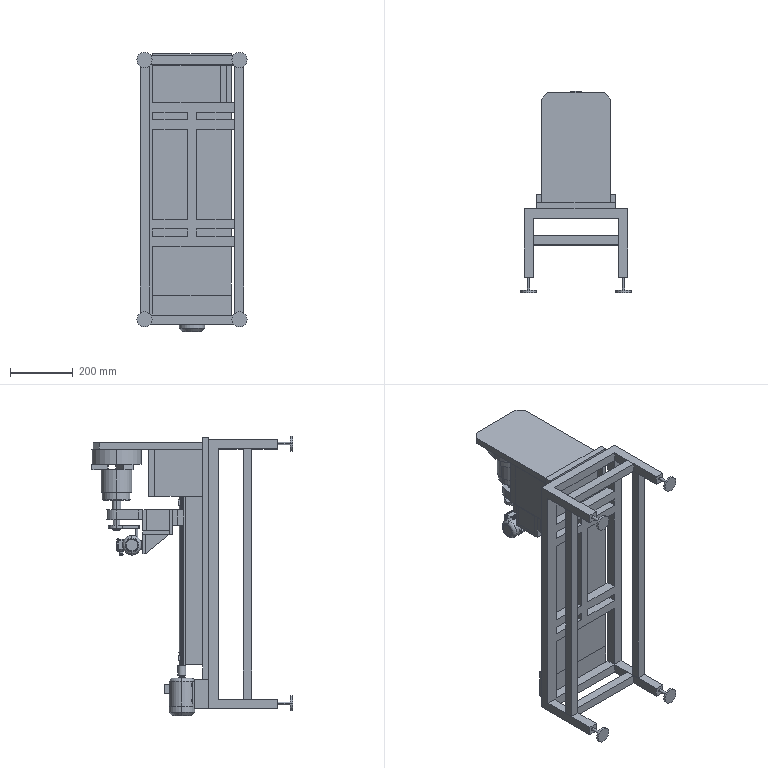Assembly | SolidWorks | mm | 29 component files | 64 solids | 2723 faces | box 351.7 x 642.03 x 891.18 mm | volume 19068992 mm3 | plane 1496 | cylinder 842 | spline 199 | cone 180 | torus 6 | commonest cylinder face diameters 5 x129 1 x116 2 x95 0.5 x65 3 x54 2.5 x27 6 x20 10 x18
Bill of materials:
BearingHousing | 1 |  | T-shaped bracket: a flat lug with a rounded end and one large through-hole, joined at right angles to a rectangular base bar that has two small through-holes.
BearingHousingFloor | 1 |  | Open-topped rectangular box-like housing. It has a thin-walled cavity, two stacked lugs with round holes sticking out from one side, a sloped flange extension with small holes on the opposite side, and stepped notches in the outline.
Belt | 1 |  | Thin-walled closed band or loop shaped like a teardrop. It has a large rounded end, a small rounded end and two straight tapering sides, with a short uniform height.
Chuck | 1 |  | Round disc with a small central through-bore. On one face is a stepped boss with split, chamfered prongs, and the bore wall shows a ridged or serrated pattern.
ChuckHolder | 1 |  | Thin sheet-like bracket: a tall flat plate with a horizontal flange at the top, a rectangular block under the flange, small side tabs, and chamfered top corners.
Coupling | 1 |  | Thick-walled cylindrical sleeve or bushing with a round through-bore and one rectangular keyway along the length of the bore.
DriveAxis | 1 |  | Slender stepped cylindrical pin or shaft: two sections of slightly different diameter, with a small rectangular slot or keyway at one end.
DriveMotor | 1 |  | Simplified cylindrical body with a domed end cap, a protruding stepped shaft, two mounting feet and a rectangular block on top. The overall envelope looks like an electric motor.
FixedFrame | 1 |  | Plain solid rectangular block (cuboid) with sharp edges and no visible holes or features.
Frame | 1 |  | Tall rectangular open frame made of square-section members, with intermediate crossbars and a central upright. It stands on four leveling-type feet, each a disc pad on a short stem.
GearedMotor | 1 |  | Detailed, roughly modelled assembly-like body: a ribbed cylindrical housing with a domed end cover and a rectangular box on top, joined through a flange to a compact angular housing that has a keyed hollow bore. The overall look resembles a motor coupled to a right-angle gearbox.
GuideRail | 1 |  | Long straight bar with a symmetric profile: V-shaped notches on both sides and rounded corners, with a row of evenly spaced small holes along one face.
LeadScrew | 1 |  | Long, slender cylindrical shaft. Both ends step down to a short section of smaller diameter.
MirrorGuideRail | 1 |  | Long straight bar with a constant cross-section. A single evenly spaced row of small holes runs along its length. The cross-section has the same notch on both sides and rounded top corners.
MirrorSlider | 1 |  | Rectangular block with a channel running all the way through it, open on the underside. The channel's internal profile has notches on both sides with rounded corners.
PolishingAxis | 1 |  | Short cylindrical pin with a raised collar of larger diameter near one end and chamfers on both ends.
PolishingHead | 1 |  | Thick circular disc with a small central through hole and a chamfer on one outer edge.
Pulley | 1 |  | Rectangular block with a channel running all the way through it, open on the underside. The channel's internal profile has notches on both sides with rounded corners.
Slider | 1 |  | Flat circular ring, like a plain washer, with a large central hole and square-edged faces.
SmallWheel | 1 |  | Thick-walled cylindrical collar or hub with a central round bore and a single rectangular keyway slot.
TRCBASHexagonThroughHoleBolt[TRCBAS3-10] | 4 |  | Hexagonal-head bolt-like part with a long plain cylindrical shank and a chamfered tip.
TRCBASHexagonThroughHoleBolt[TRCBAS5-10] | 4 |  | Hexagonal-head bolt-like part with a shorter plain cylindrical shank and a chamfered tip.
Workpiece | 1 |  | Thin-walled cylindrical tube or sleeve, open at both ends.
Mates:
1. coincident | Pulley-1 face at (0, 0, -195) dir (0, 0, 1) | SmallWheel-1 face at (48.507, -64.609, -195) dir (0, 0, 1)
2. concentric | LeadScrew-1 face at (0, -208.707, -601) dir (0, 0, -1) r 8 | DriveMotor-1 face at (0, -208.707, -654.301) dir (0, 0, -1) r 5.5
3. concentric | DriveMotor-1 face at (0, -208.707, -654.301) dir (0, 0, -1) r 5.5 | Coupling-1 face at (0, -208.707, -643.144) dir (0, 0, -1) r 12.5
4. coincident | DriveMotor-1 face at (1.5, -209.324, -655.301) dir (1, 0, 0) | Coupling-1 face at (1.5, -205.207, -653.144) dir (-1, 0, 0)
5. distance | DriveMotor-1 face at (19.858, -243.43, -695.801) dir (0, 0, 1) | FixedFrame-1 face at (125, -251.035, -685.801) dir (0, 0, 1)
6. concentric | SmallWheel-1 face at (48.507, -64.609, -205) dir (0, 0, 1) r 7.5 | GearedMotor-1 face at (48.507, -64.609, -274.5) dir (0, 0, 1) r 3.5
7. coincident | BearingHousingFloor-1 face at (68.507, -84.609, -286.341) dir (0, 1, 0) | GearedMotor-1 face at (58.507, -84.609, -272.25) dir (0, -1, 0)
8. concentric | GearedMotor-1 face at (48.507, -64.609, -274.5) dir (0, 0, 1) r 3.5 | DriveAxis-1 face at (48.507, -64.609, -242) dir (0, 0, -1) r 3.5
9. coincident | GearedMotor-1 face at (47.257, -61.339, -275) dir (1, 0, 0) | DriveAxis-1 face at (47.257, -62.109, -243.502) dir (1, 0, 0)
10. coincident | GearedMotor-1 face at (42.688, -58.79, -275) dir (0, 0, -1) | DriveAxis-1 face at (48.507, -64.609, -275) dir (0, 0, -1)
11. coincident | SmallWheel-1 face at (48.507, -64.609, -195) dir (0, 0, 1) | DriveAxis-1 face at (48.507, -64.609, -195) dir (0, 0, 1)
12. concentric | GearedMotor-1 face at (62.257, -81.609, -269.75) dir (0, -1, 0) r 1.625 | TRCBASHexagonThroughHoleBolt[TRCBAS3-10]-1 face at (62.257, -79.609, -269.75) dir (0, 1, 0) r 1.5
13. coincident | GearedMotor-1 face at (50.603, -81.609, -272.25) dir (0, 1, 0) | TRCBASHexagonThroughHoleBolt[TRCBAS3-10]-1 face at (65.003, -81.609, -269.608) dir (0, -1, 0)
14. concentric | GearedMotor-1 face at (34.757, -81.609, -269.75) dir (0, -1, 0) r 1.625 | TRCBASHexagonThroughHoleBolt[TRCBAS3-10]-2 face at (34.757, -79.609, -269.75) dir (0, 1, 0) r 1.5
15. coincident | GearedMotor-1 face at (31.257, -81.609, -272.25) dir (0, 1, 0) | TRCBASHexagonThroughHoleBolt[TRCBAS3-10]-2 face at (37.507, -81.609, -269.75) dir (0, -1, 0)
16. concentric | GearedMotor-1 face at (62.257, -81.609, -247.25) dir (0, -1, 0) r 1.625 | TRCBASHexagonThroughHoleBolt[TRCBAS3-10]-3 face at (62.257, -79.609, -247.25) dir (0, 1, 0) r 1.5
17. coincident | GearedMotor-1 face at (50.603, -81.609, -250.5) dir (0, 1, 0) | TRCBASHexagonThroughHoleBolt[TRCBAS3-10]-3 face at (65.003, -81.609, -247.108) dir (0, -1, 0)
18. concentric | GearedMotor-1 face at (34.757, -81.609, -247.25) dir (0, -1, 0) r 1.625 | TRCBASHexagonThroughHoleBolt[TRCBAS3-10]-4 face at (34.757, -79.609, -247.25) dir (0, 1, 0) r 1.5
19. coincident | GearedMotor-1 face at (31.257, -81.609, -250.5) dir (0, 1, 0) | TRCBASHexagonThroughHoleBolt[TRCBAS3-10]-4 face at (37.503, -81.609, -247.108) dir (0, -1, 0)
20. concentric | DriveMotor-1 edge at (31.25, -244.207, -754.301) dir (0, 1, 0) r 2.5 | TRCBASHexagonThroughHoleBolt[TRCBAS5-10]-1 face at (31.25, -240.707, -754.301) dir (0, 1, 0) r 2.5
21. parallel | DriveMotor-1 face at (27, -244.207, -763.301) dir (0, 1, 0) | FixedFrame-1 face at (0, -248.735, 48) dir (0, 1, 0)
22. coincident | DriveMotor-1 face at (27, -244.207, -763.301) dir (0, 1, 0) | TRCBASHexagonThroughHoleBolt[TRCBAS5-10]-1 face at (34.621, -244.207, -756.454) dir (0, -1, 0)
23. concentric | DriveMotor-1 face at (31.25, -249.207, -704.301) dir (0, 1, 0) r 2.5 | TRCBASHexagonThroughHoleBolt[TRCBAS5-10]-2 face at (31.25, -240.707, -704.301) dir (0, 1, 0) r 2.5
24. coincident | DriveMotor-1 face at (27, -244.207, -763.301) dir (0, 1, 0) | TRCBASHexagonThroughHoleBolt[TRCBAS5-10]-2 face at (34.621, -244.207, -706.454) dir (0, -1, 0)
25. concentric | DriveMotor-1 face at (-31.25, -249.207, -704.301) dir (0, 1, 0) r 2.5 | TRCBASHexagonThroughHoleBolt[TRCBAS5-10]-3 face at (-31.25, -240.707, -704.301) dir (0, 1, 0) r 2.5
26. coincident | DriveMotor-1 face at (-27, -244.207, -763.301) dir (0, 1, 0) | TRCBASHexagonThroughHoleBolt[TRCBAS5-10]-3 face at (-27.879, -244.207, -706.454) dir (0, -1, 0)
27. concentric | DriveMotor-1 face at (-31.25, -249.207, -754.301) dir (0, 1, 0) r 2.5 | TRCBASHexagonThroughHoleBolt[TRCBAS5-10]-4 face at (-31.25, -240.707, -754.301) dir (0, 1, 0) r 2.5
28. coincident | DriveMotor-1 face at (-27, -244.207, -763.301) dir (0, 1, 0) | TRCBASHexagonThroughHoleBolt[TRCBAS5-10]-4 face at (-27.879, -244.207, -756.454) dir (0, -1, 0)